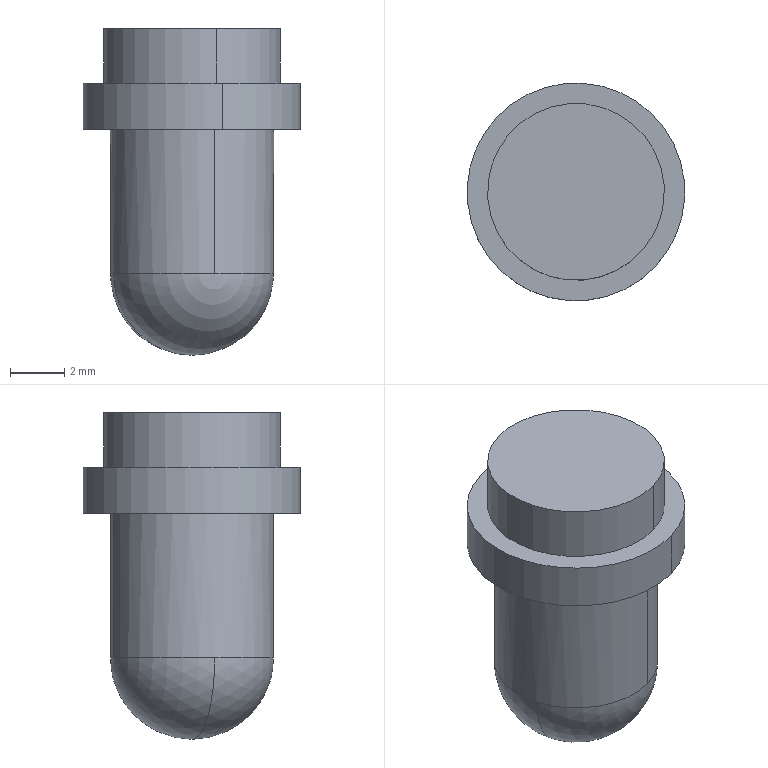Component | SolidWorks | LeftDoorAssembly-1_Pin-1 | 1 solid | 11 faces | box 8 x 8 x 12 mm | volume 358 mm3 | cylinder 6 | plane 3 | sphere 2 | commonest cylinder face diameters 6 x2 8 x2 6.5 x2
build123d program:
from build123d import *


with BuildPart() as part:
    # Sketch1 → Revolve1 (revolve)
    with BuildSketch(Plane.XY, mode=Mode.PRIVATE) as revolve1_sk:
        with BuildLine():
            Line((0, 0), (3.25, 0))
            Line((3.25, 0), (3.25, 2))
            Line((3.25, 2), (4, 2))
            Line((4, 2), (4, 3.7))
            Line((4, 3.7), (3, 3.7))
            Line((3, 3.7), (3, 9))
            ThreePointArc((3, 9), (2.121, 11.121), (0, 12))
            Line((0, 12), (0, 0))
        make_face()
    revolve(revolve1_sk.sketch.rotate(Axis((0, 0, 0), (0, 1, 0)), 90), axis=Axis((0, 0, 0), (0, 1, 0)))


solid = part.part

# Placed as in the assembly
solid = solid.moved(Location((275.828, 196.273, 72.2), (-90, 0, 0)))
STEP:
#1=CARTESIAN_POINT('',(10.859,7.727,2.37));
#2=VERTEX_POINT('',#1);
#3=CARTESIAN_POINT('',(10.746,7.694,2.488));
#4=VERTEX_POINT('',#3);
#5=CARTESIAN_POINT('',(10.859,7.727,2.488));
#6=DIRECTION('',(-0.2786,0.9604,-0.));
#7=DIRECTION('',(-0.9604,-0.2786,0.));
#8=AXIS2_PLACEMENT_3D('',#5,#6,#7);
#9=CIRCLE('',#8,0.1181);
#10=EDGE_CURVE('',#2,#4,#9,.T.);
#11=ORIENTED_EDGE('',*,*,#10,.F.);
#12=CARTESIAN_POINT('',(10.973,7.76,2.488));
#13=VERTEX_POINT('',#12);
#14=CARTESIAN_POINT('',(10.859,7.727,2.488));
#15=DIRECTION('',(0.2786,-0.9604,0.));
#16=DIRECTION('',(0.9604,0.2786,0.));
#17=AXIS2_PLACEMENT_3D('',#14,#15,#16);
#18=CIRCLE('',#17,0.1181);
#19=EDGE_CURVE('',#2,#13,#18,.T.);
#20=ORIENTED_EDGE('',*,*,#19,.T.);
#21=CARTESIAN_POINT('',(10.892,7.614,2.488));
#22=VERTEX_POINT('',#21);
#23=CARTESIAN_POINT('',(10.859,7.727,2.488));
#24=DIRECTION('',(-0.,0.,1.));
#25=DIRECTION('',(-0.2786,0.9604,0.));
#26=AXIS2_PLACEMENT_3D('',#23,#24,#25);
#27=CIRCLE('',#26,0.1181);
#28=EDGE_CURVE('',#22,#13,#27,.T.);
#29=ORIENTED_EDGE('',*,*,#28,.F.);
#30=CARTESIAN_POINT('',(10.859,7.727,2.488));
#31=DIRECTION('',(-0.,0.,1.));
#32=DIRECTION('',(-0.2786,0.9604,0.));
#33=AXIS2_PLACEMENT_3D('',#30,#31,#32);
#34=CIRCLE('',#33,0.1181);
#35=EDGE_CURVE('',#4,#22,#34,.T.);
#36=ORIENTED_EDGE('',*,*,#35,.F.);
#37=EDGE_LOOP('',(#11,#20,#29,#36));
#38=FACE_OUTER_BOUND('',#37,.T.);
#39=CARTESIAN_POINT('',(10.859,7.727,2.488));
#40=DIRECTION('',(0.2786,-0.9604,0.));
#41=DIRECTION('',(-0.9604,-0.2786,-0.));
#42=AXIS2_PLACEMENT_3D('',#39,#40,#41);
#43=SPHERICAL_SURFACE('',#42,0.1181);
#44=ADVANCED_FACE('',(#38),#43,.T.);
#45=CARTESIAN_POINT('',(10.826,7.841,2.488));
#46=VERTEX_POINT('',#45);
#47=CARTESIAN_POINT('',(10.859,7.727,2.488));
#48=DIRECTION('',(-0.,0.,1.));
#49=DIRECTION('',(-0.2786,0.9604,0.));
#50=AXIS2_PLACEMENT_3D('',#47,#48,#49);
#51=CIRCLE('',#50,0.1181);
#52=EDGE_CURVE('',#46,#4,#51,.T.);
#53=ORIENTED_EDGE('',*,*,#52,.T.);
#54=ORIENTED_EDGE('',*,*,#35,.T.);
#55=CARTESIAN_POINT('',(10.892,7.614,2.697));
#56=VERTEX_POINT('',#55);
#57=CARTESIAN_POINT('',(10.892,7.614,2.843));
#58=DIRECTION('',(-0.,0.,1.));
#59=VECTOR('',#58,39.37);
#60=LINE('',#57,#59);
#61=EDGE_CURVE('',#22,#56,#60,.T.);
#62=ORIENTED_EDGE('',*,*,#61,.T.);
#63=CARTESIAN_POINT('',(10.826,7.841,2.697));
#64=VERTEX_POINT('',#63);
#65=CARTESIAN_POINT('',(10.859,7.727,2.697));
#66=DIRECTION('',(-0.,0.,1.));
#67=DIRECTION('',(-0.2786,0.9604,0.));
#68=AXIS2_PLACEMENT_3D('',#65,#66,#67);
#69=CIRCLE('',#68,0.1181);
#70=EDGE_CURVE('',#64,#56,#69,.T.);
#71=ORIENTED_EDGE('',*,*,#70,.F.);
#72=CARTESIAN_POINT('',(10.826,7.841,2.843));
#73=DIRECTION('',(-0.,0.,1.));
#74=VECTOR('',#73,39.37);
#75=LINE('',#72,#74);
#76=EDGE_CURVE('',#46,#64,#75,.T.);
#77=ORIENTED_EDGE('',*,*,#76,.F.);
#78=EDGE_LOOP('',(#53,#54,#62,#71,#77));
#79=FACE_OUTER_BOUND('',#78,.T.);
#80=CARTESIAN_POINT('',(10.859,7.727,2.843));
#81=DIRECTION('',(-0.,0.,1.));
#82=DIRECTION('',(-0.2786,0.9604,0.));
#83=AXIS2_PLACEMENT_3D('',#80,#81,#82);
#84=CYLINDRICAL_SURFACE('',#83,0.1181);
#85=ADVANCED_FACE('',(#79),#84,.T.);
#86=CARTESIAN_POINT('',(10.815,7.879,2.697));
#87=VERTEX_POINT('',#86);
#88=CARTESIAN_POINT('',(10.903,7.576,2.697));
#89=VERTEX_POINT('',#88);
#90=CARTESIAN_POINT('',(10.859,7.727,2.697));
#91=DIRECTION('',(-0.,0.,1.));
#92=DIRECTION('',(-0.2786,0.9604,-0.));
#93=AXIS2_PLACEMENT_3D('',#90,#91,#92);
#94=CIRCLE('',#93,0.1575);
#95=EDGE_CURVE('',#87,#89,#94,.T.);
#96=ORIENTED_EDGE('',*,*,#95,.T.);
#97=CARTESIAN_POINT('',(10.903,7.576,2.764));
#98=VERTEX_POINT('',#97);
#99=CARTESIAN_POINT('',(10.903,7.576,2.843));
#100=DIRECTION('',(-0.,0.,1.));
#101=VECTOR('',#100,39.37);
#102=LINE('',#99,#101);
#103=EDGE_CURVE('',#89,#98,#102,.T.);
#104=ORIENTED_EDGE('',*,*,#103,.T.);
#105=CARTESIAN_POINT('',(10.815,7.879,2.764));
#106=VERTEX_POINT('',#105);
#107=CARTESIAN_POINT('',(10.859,7.727,2.764));
#108=DIRECTION('',(-0.,0.,1.));
#109=DIRECTION('',(-0.2786,0.9604,-0.));
#110=AXIS2_PLACEMENT_3D('',#107,#108,#109);
#111=CIRCLE('',#110,0.1575);
#112=EDGE_CURVE('',#106,#98,#111,.T.);
#113=ORIENTED_EDGE('',*,*,#112,.F.);
#114=CARTESIAN_POINT('',(10.815,7.879,2.843));
#115=DIRECTION('',(-0.,0.,1.));
#116=VECTOR('',#115,39.37);
#117=LINE('',#114,#116);
#118=EDGE_CURVE('',#87,#106,#117,.T.);
#119=ORIENTED_EDGE('',*,*,#118,.F.);
#120=EDGE_LOOP('',(#96,#104,#113,#119));
#121=FACE_OUTER_BOUND('',#120,.T.);
#122=CARTESIAN_POINT('',(10.859,7.727,2.843));
#123=DIRECTION('',(-0.,0.,1.));
#124=DIRECTION('',(-0.2786,0.9604,-0.));
#125=AXIS2_PLACEMENT_3D('',#122,#123,#124);
#126=CYLINDRICAL_SURFACE('',#125,0.1575);
#127=ADVANCED_FACE('',(#121),#126,.T.);
#128=CARTESIAN_POINT('',(10.824,7.85,2.764));
#129=VERTEX_POINT('',#128);
#130=CARTESIAN_POINT('',(10.895,7.604,2.764));
#131=VERTEX_POINT('',#130);
#132=CARTESIAN_POINT('',(10.859,7.727,2.764));
#133=DIRECTION('',(-0.,0.,1.));
#134=DIRECTION('',(-0.2786,0.9604,0.));
#135=AXIS2_PLACEMENT_3D('',#132,#133,#134);
#136=CIRCLE('',#135,0.128);
#137=EDGE_CURVE('',#129,#131,#136,.T.);
#138=ORIENTED_EDGE('',*,*,#137,.T.);
#139=CARTESIAN_POINT('',(10.895,7.604,2.843));
#140=VERTEX_POINT('',#139);
#141=CARTESIAN_POINT('',(10.895,7.604,2.843));
#142=DIRECTION('',(-0.,0.,1.));
#143=VECTOR('',#142,39.37);
#144=LINE('',#141,#143);
#145=EDGE_CURVE('',#131,#140,#144,.T.);
#146=ORIENTED_EDGE('',*,*,#145,.T.);
#147=CARTESIAN_POINT('',(10.824,7.85,2.843));
#148=VERTEX_POINT('',#147);
#149=CARTESIAN_POINT('',(10.859,7.727,2.843));
#150=DIRECTION('',(-0.,0.,1.));
#151=DIRECTION('',(-0.2786,0.9604,0.));
#152=AXIS2_PLACEMENT_3D('',#149,#150,#151);
#153=CIRCLE('',#152,0.128);
#154=EDGE_CURVE('',#148,#140,#153,.T.);
#155=ORIENTED_EDGE('',*,*,#154,.F.);
#156=CARTESIAN_POINT('',(10.824,7.85,2.843));
#157=DIRECTION('',(-0.,0.,1.));
#158=VECTOR('',#157,39.37);
#159=LINE('',#156,#158);
#160=EDGE_CURVE('',#129,#148,#159,.T.);
#161=ORIENTED_EDGE('',*,*,#160,.F.);
#162=EDGE_LOOP('',(#138,#146,#155,#161));
#163=FACE_OUTER_BOUND('',#162,.T.);
#164=CARTESIAN_POINT('',(10.859,7.727,2.843));
#165=DIRECTION('',(-0.,0.,1.));
#166=DIRECTION('',(-0.2786,0.9604,0.));
#167=AXIS2_PLACEMENT_3D('',#164,#165,#166);
#168=CYLINDRICAL_SURFACE('',#167,0.128);
#169=ADVANCED_FACE('',(#163),#168,.T.);
#170=ORIENTED_EDGE('',*,*,#154,.T.);
#171=CARTESIAN_POINT('',(10.859,7.727,2.843));
#172=DIRECTION('',(-0.,0.,1.));
#173=DIRECTION('',(-0.2786,0.9604,0.));
#174=AXIS2_PLACEMENT_3D('',#171,#172,#173);
#175=CIRCLE('',#174,0.128);
#176=EDGE_CURVE('',#140,#148,#175,.T.);
#177=ORIENTED_EDGE('',*,*,#176,.T.);
#178=EDGE_LOOP('',(#170,#177));
#179=FACE_OUTER_BOUND('',#178,.T.);
#180=CARTESIAN_POINT('',(10.859,7.727,2.843));
#181=DIRECTION('',(-0.,0.,1.));
#182=DIRECTION('',(-0.2786,0.9604,-0.));
#183=AXIS2_PLACEMENT_3D('',#180,#181,#182);
#184=PLANE('',#183);
#185=ADVANCED_FACE('',(#179),#184,.T.);
#186=ORIENTED_EDGE('',*,*,#145,.F.);
#187=CARTESIAN_POINT('',(10.859,7.727,2.764));
#188=DIRECTION('',(-0.,0.,1.));
#189=DIRECTION('',(-0.2786,0.9604,0.));
#190=AXIS2_PLACEMENT_3D('',#187,#188,#189);
#191=CIRCLE('',#190,0.128);
#192=EDGE_CURVE('',#131,#129,#191,.T.);
#193=ORIENTED_EDGE('',*,*,#192,.T.);
#194=ORIENTED_EDGE('',*,*,#160,.T.);
#195=ORIENTED_EDGE('',*,*,#176,.F.);
#196=EDGE_LOOP('',(#186,#193,#194,#195));
#197=FACE_OUTER_BOUND('',#196,.T.);
#198=CARTESIAN_POINT('',(10.859,7.727,2.843));
#199=DIRECTION('',(-0.,0.,1.));
#200=DIRECTION('',(-0.2786,0.9604,0.));
#201=AXIS2_PLACEMENT_3D('',#198,#199,#200);
#202=CYLINDRICAL_SURFACE('',#201,0.128);
#203=ADVANCED_FACE('',(#197),#202,.T.);
#204=ORIENTED_EDGE('',*,*,#112,.T.);
#205=CARTESIAN_POINT('',(10.859,7.727,2.764));
#206=DIRECTION('',(-0.,0.,1.));
#207=DIRECTION('',(-0.2786,0.9604,-0.));
#208=AXIS2_PLACEMENT_3D('',#205,#206,#207);
#209=CIRCLE('',#208,0.1575);
#210=EDGE_CURVE('',#98,#106,#209,.T.);
#211=ORIENTED_EDGE('',*,*,#210,.T.);
#212=EDGE_LOOP('',(#204,#211));
#213=FACE_OUTER_BOUND('',#212,.T.);
#214=ORIENTED_EDGE('',*,*,#137,.F.);
#215=ORIENTED_EDGE('',*,*,#192,.F.);
#216=EDGE_LOOP('',(#214,#215));
#217=FACE_BOUND('',#216,.T.);
#218=CARTESIAN_POINT('',(10.859,7.727,2.764));
#219=DIRECTION('',(-0.,0.,1.));
#220=DIRECTION('',(-0.2786,0.9604,-0.));
#221=AXIS2_PLACEMENT_3D('',#218,#219,#220);
#222=PLANE('',#221);
#223=ADVANCED_FACE('',(#213,#217),#222,.T.);
#224=ORIENTED_EDGE('',*,*,#103,.F.);
#225=CARTESIAN_POINT('',(10.859,7.727,2.697));
#226=DIRECTION('',(-0.,0.,1.));
#227=DIRECTION('',(-0.2786,0.9604,-0.));
#228=AXIS2_PLACEMENT_3D('',#225,#226,#227);
#229=CIRCLE('',#228,0.1575);
#230=EDGE_CURVE('',#89,#87,#229,.T.);
#231=ORIENTED_EDGE('',*,*,#230,.T.);
#232=ORIENTED_EDGE('',*,*,#118,.T.);
#233=ORIENTED_EDGE('',*,*,#210,.F.);
#234=EDGE_LOOP('',(#224,#231,#232,#233));
#235=FACE_OUTER_BOUND('',#234,.T.);
#236=CARTESIAN_POINT('',(10.859,7.727,2.843));
#237=DIRECTION('',(-0.,0.,1.));
#238=DIRECTION('',(-0.2786,0.9604,-0.));
#239=AXIS2_PLACEMENT_3D('',#236,#237,#238);
#240=CYLINDRICAL_SURFACE('',#239,0.1575);
#241=ADVANCED_FACE('',(#235),#240,.T.);
#242=ORIENTED_EDGE('',*,*,#70,.T.);
#243=CARTESIAN_POINT('',(10.859,7.727,2.697));
#244=DIRECTION('',(-0.,0.,1.));
#245=DIRECTION('',(-0.2786,0.9604,0.));
#246=AXIS2_PLACEMENT_3D('',#243,#244,#245);
#247=CIRCLE('',#246,0.1181);
#248=EDGE_CURVE('',#56,#64,#247,.T.);
#249=ORIENTED_EDGE('',*,*,#248,.T.);
#250=EDGE_LOOP('',(#242,#249));
#251=FACE_BOUND('',#250,.T.);
#252=ORIENTED_EDGE('',*,*,#95,.F.);
#253=ORIENTED_EDGE('',*,*,#230,.F.);
#254=EDGE_LOOP('',(#252,#253));
#255=FACE_OUTER_BOUND('',#254,.T.);
#256=CARTESIAN_POINT('',(10.859,7.727,2.697));
#257=DIRECTION('',(0.,-0.,-1.));
#258=DIRECTION('',(0.2786,-0.9604,0.));
#259=AXIS2_PLACEMENT_3D('',#256,#257,#258);
#260=PLANE('',#259);
#261=ADVANCED_FACE('',(#251,#255),#260,.T.);
#262=ORIENTED_EDGE('',*,*,#61,.F.);
#263=ORIENTED_EDGE('',*,*,#28,.T.);
#264=CARTESIAN_POINT('',(10.859,7.727,2.488));
#265=DIRECTION('',(-0.,0.,1.));
#266=DIRECTION('',(-0.2786,0.9604,0.));
#267=AXIS2_PLACEMENT_3D('',#264,#265,#266);
#268=CIRCLE('',#267,0.1181);
#269=EDGE_CURVE('',#13,#46,#268,.T.);
#270=ORIENTED_EDGE('',*,*,#269,.T.);
#271=ORIENTED_EDGE('',*,*,#76,.T.);
#272=ORIENTED_EDGE('',*,*,#248,.F.);
#273=EDGE_LOOP('',(#262,#263,#270,#271,#272));
#274=FACE_OUTER_BOUND('',#273,.T.);
#275=CARTESIAN_POINT('',(10.859,7.727,2.843));
#276=DIRECTION('',(-0.,0.,1.));
#277=DIRECTION('',(-0.2786,0.9604,0.));
#278=AXIS2_PLACEMENT_3D('',#275,#276,#277);
#279=CYLINDRICAL_SURFACE('',#278,0.1181);
#280=ADVANCED_FACE('',(#274),#279,.T.);
#281=ORIENTED_EDGE('',*,*,#19,.F.);
#282=ORIENTED_EDGE('',*,*,#10,.T.);
#283=ORIENTED_EDGE('',*,*,#52,.F.);
#284=ORIENTED_EDGE('',*,*,#269,.F.);
#285=EDGE_LOOP('',(#281,#282,#283,#284));
#286=FACE_OUTER_BOUND('',#285,.T.);
#287=CARTESIAN_POINT('',(10.859,7.727,2.488));
#288=DIRECTION('',(0.2786,-0.9604,0.));
#289=DIRECTION('',(-0.9604,-0.2786,-0.));
#290=AXIS2_PLACEMENT_3D('',#287,#288,#289);
#291=SPHERICAL_SURFACE('',#290,0.1181);
#292=ADVANCED_FACE('',(#286),#291,.T.);
#293=CLOSED_SHELL('',(#44,#85,#127,#169,#185,#203,#223,#241,#261,#280,#292));
#294=MANIFOLD_SOLID_BREP('',#293);
#295=CARTESIAN_POINT('',(0.,0.,0.));
#296=DIRECTION('',(0.,0.,1.));
#297=DIRECTION('',(1.,0.,0.));
#298=AXIS2_PLACEMENT_3D('',#295,#296,#297);
#299=(LENGTH_UNIT()NAMED_UNIT(*)SI_UNIT($,.METRE.));
#300=LENGTH_MEASURE_WITH_UNIT(LENGTH_MEASURE(0.0254),#299);
#301=DIMENSIONAL_EXPONENTS(1.,0.,0.,0.,0.,0.,0.);
#302=(CONVERSION_BASED_UNIT('',#300)LENGTH_UNIT()NAMED_UNIT(#301));
#303=UNCERTAINTY_MEASURE_WITH_UNIT(LENGTH_MEASURE(0.00001),#302,'','');
#304=(NAMED_UNIT(*)PLANE_ANGLE_UNIT()SI_UNIT($,.RADIAN.));
#305=(NAMED_UNIT(*)SI_UNIT($,.STERADIAN.)SOLID_ANGLE_UNIT());
#306=(GEOMETRIC_REPRESENTATION_CONTEXT(3)GLOBAL_UNCERTAINTY_ASSIGNED_CONTEXT((#303))GLOBAL_UNIT_ASSIGNED_CONTEXT((#302,#304,#305))REPRESENTATION_CONTEXT('',''));
#307=ADVANCED_BREP_SHAPE_REPRESENTATION('',(#294,#298),#306);
#308=COLOUR_RGB('',0.7922,0.8196,0.9333);
#309=FILL_AREA_STYLE_COLOUR('',#308);
#310=FILL_AREA_STYLE('',(#309));
#311=SURFACE_STYLE_FILL_AREA(#310);
#312=SURFACE_SIDE_STYLE('',(#311));
#313=SURFACE_STYLE_USAGE(.BOTH.,#312);
#314=PRESENTATION_STYLE_ASSIGNMENT((#313));
#315=STYLED_ITEM('',(#314),#294);
#316=PRESENTATION_LAYER_ASSIGNMENT('','',(#315));
#317=(LENGTH_UNIT()NAMED_UNIT(*)SI_UNIT($,.METRE.));
#318=LENGTH_MEASURE_WITH_UNIT(LENGTH_MEASURE(0.0254),#317);
#319=DIMENSIONAL_EXPONENTS(1.,0.,0.,0.,0.,0.,0.);
#320=(CONVERSION_BASED_UNIT('',#318)LENGTH_UNIT()NAMED_UNIT(#319));
#321=UNCERTAINTY_MEASURE_WITH_UNIT(LENGTH_MEASURE(0.00001),#320,'','');
#322=(NAMED_UNIT(*)PLANE_ANGLE_UNIT()SI_UNIT($,.RADIAN.));
#323=(NAMED_UNIT(*)SI_UNIT($,.STERADIAN.)SOLID_ANGLE_UNIT());
#324=(GEOMETRIC_REPRESENTATION_CONTEXT(3)GLOBAL_UNCERTAINTY_ASSIGNED_CONTEXT((#321))GLOBAL_UNIT_ASSIGNED_CONTEXT((#320,#322,#323))REPRESENTATION_CONTEXT('',''));
#325=MECHANICAL_DESIGN_GEOMETRIC_PRESENTATION_REPRESENTATION('',(#315),#324);